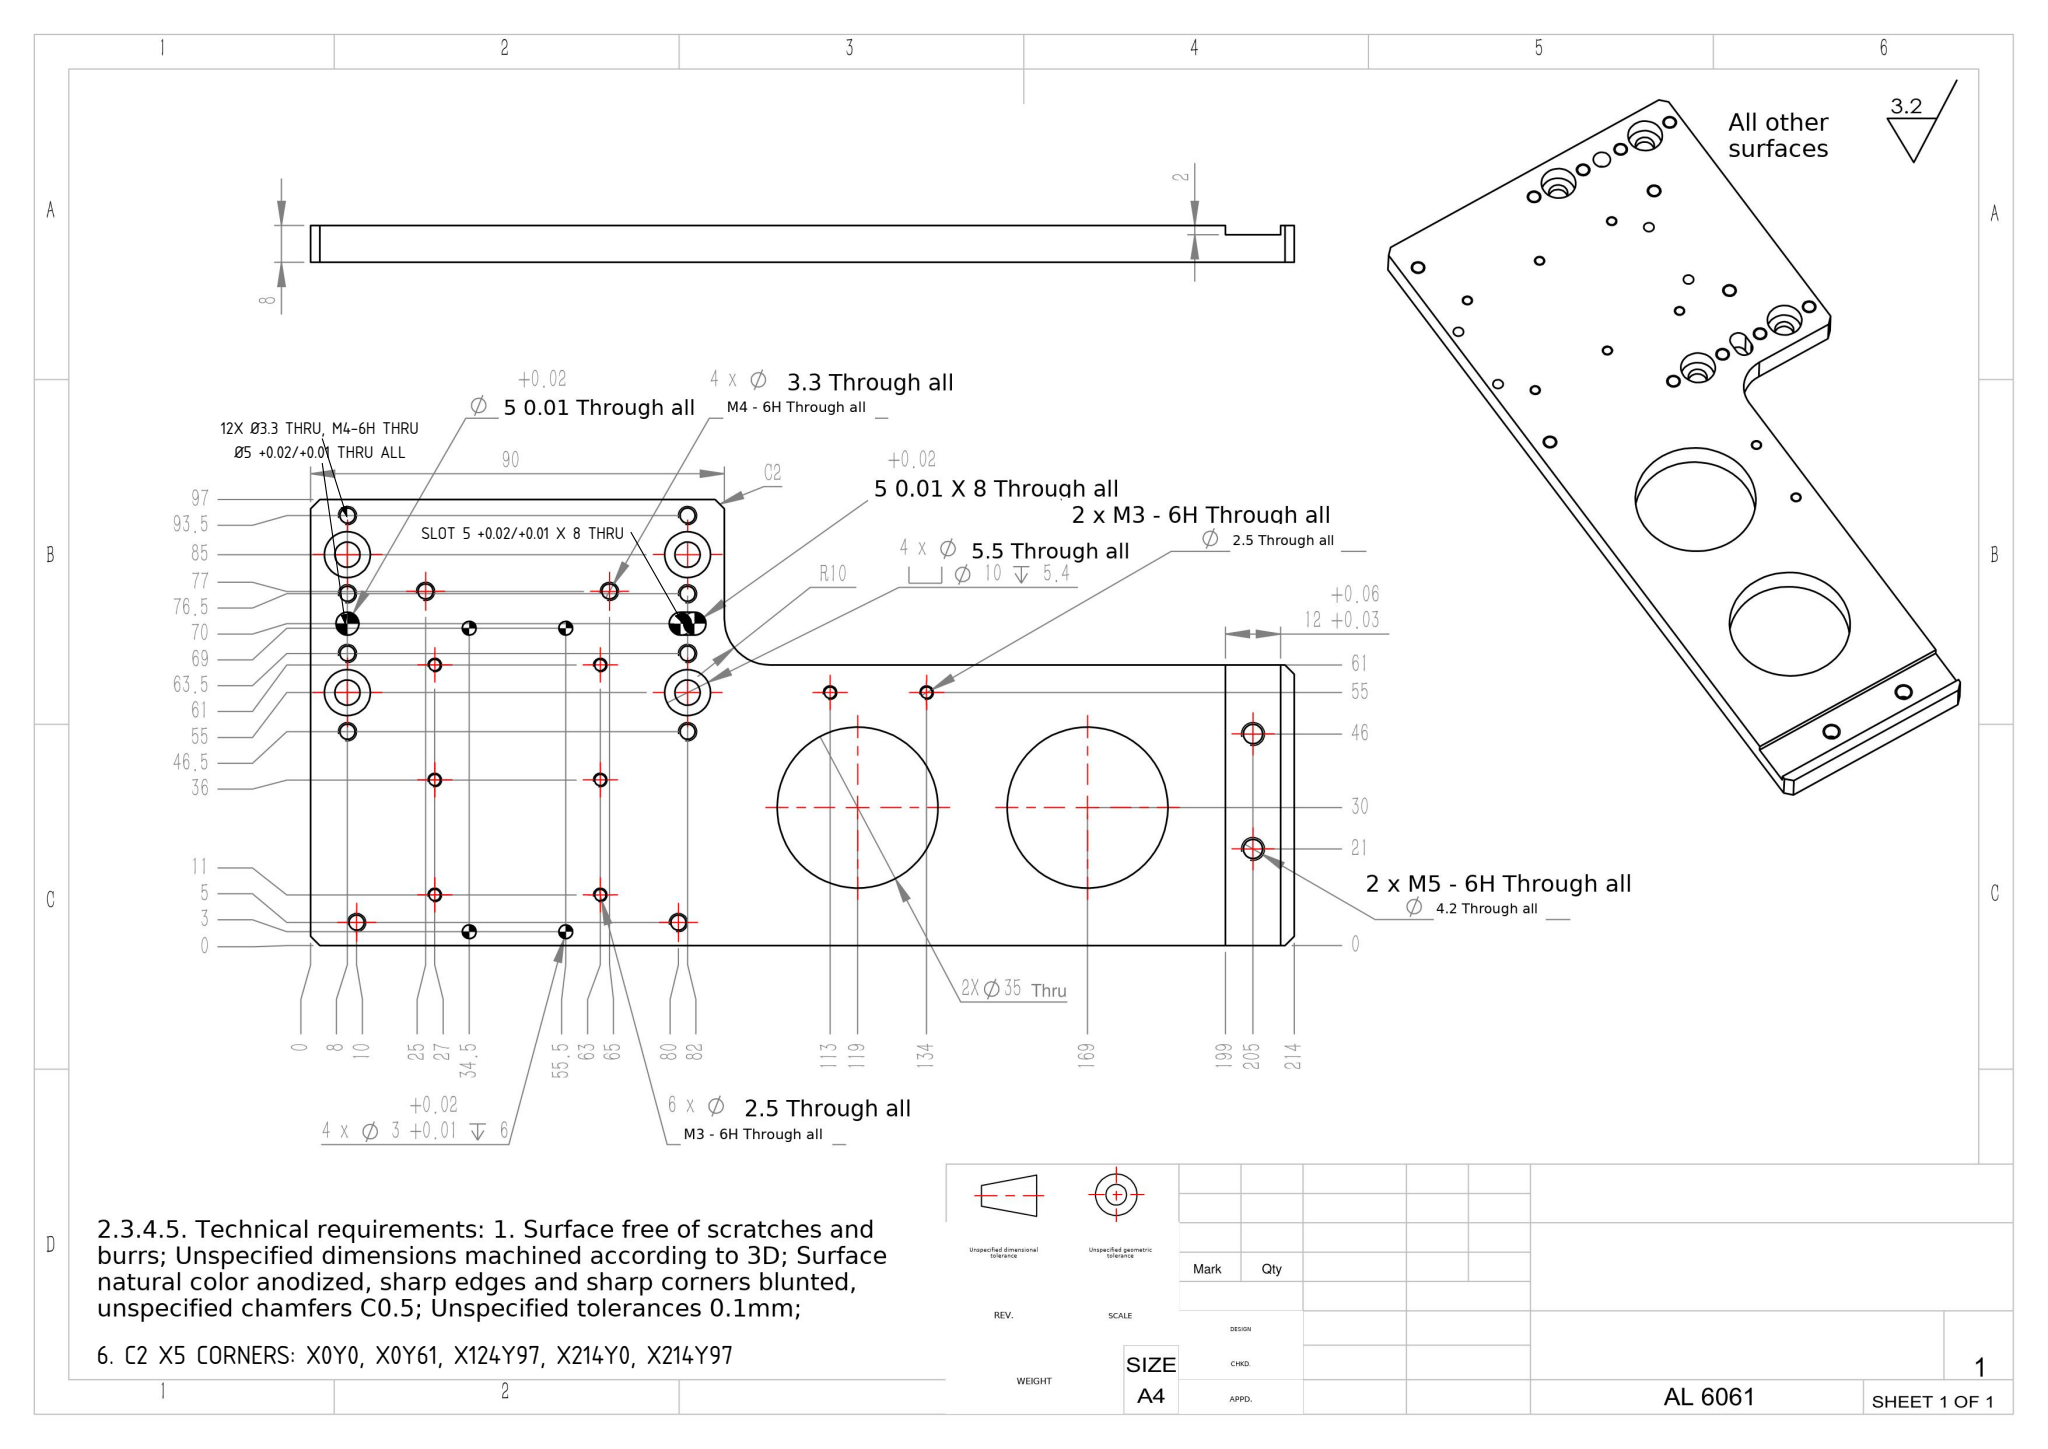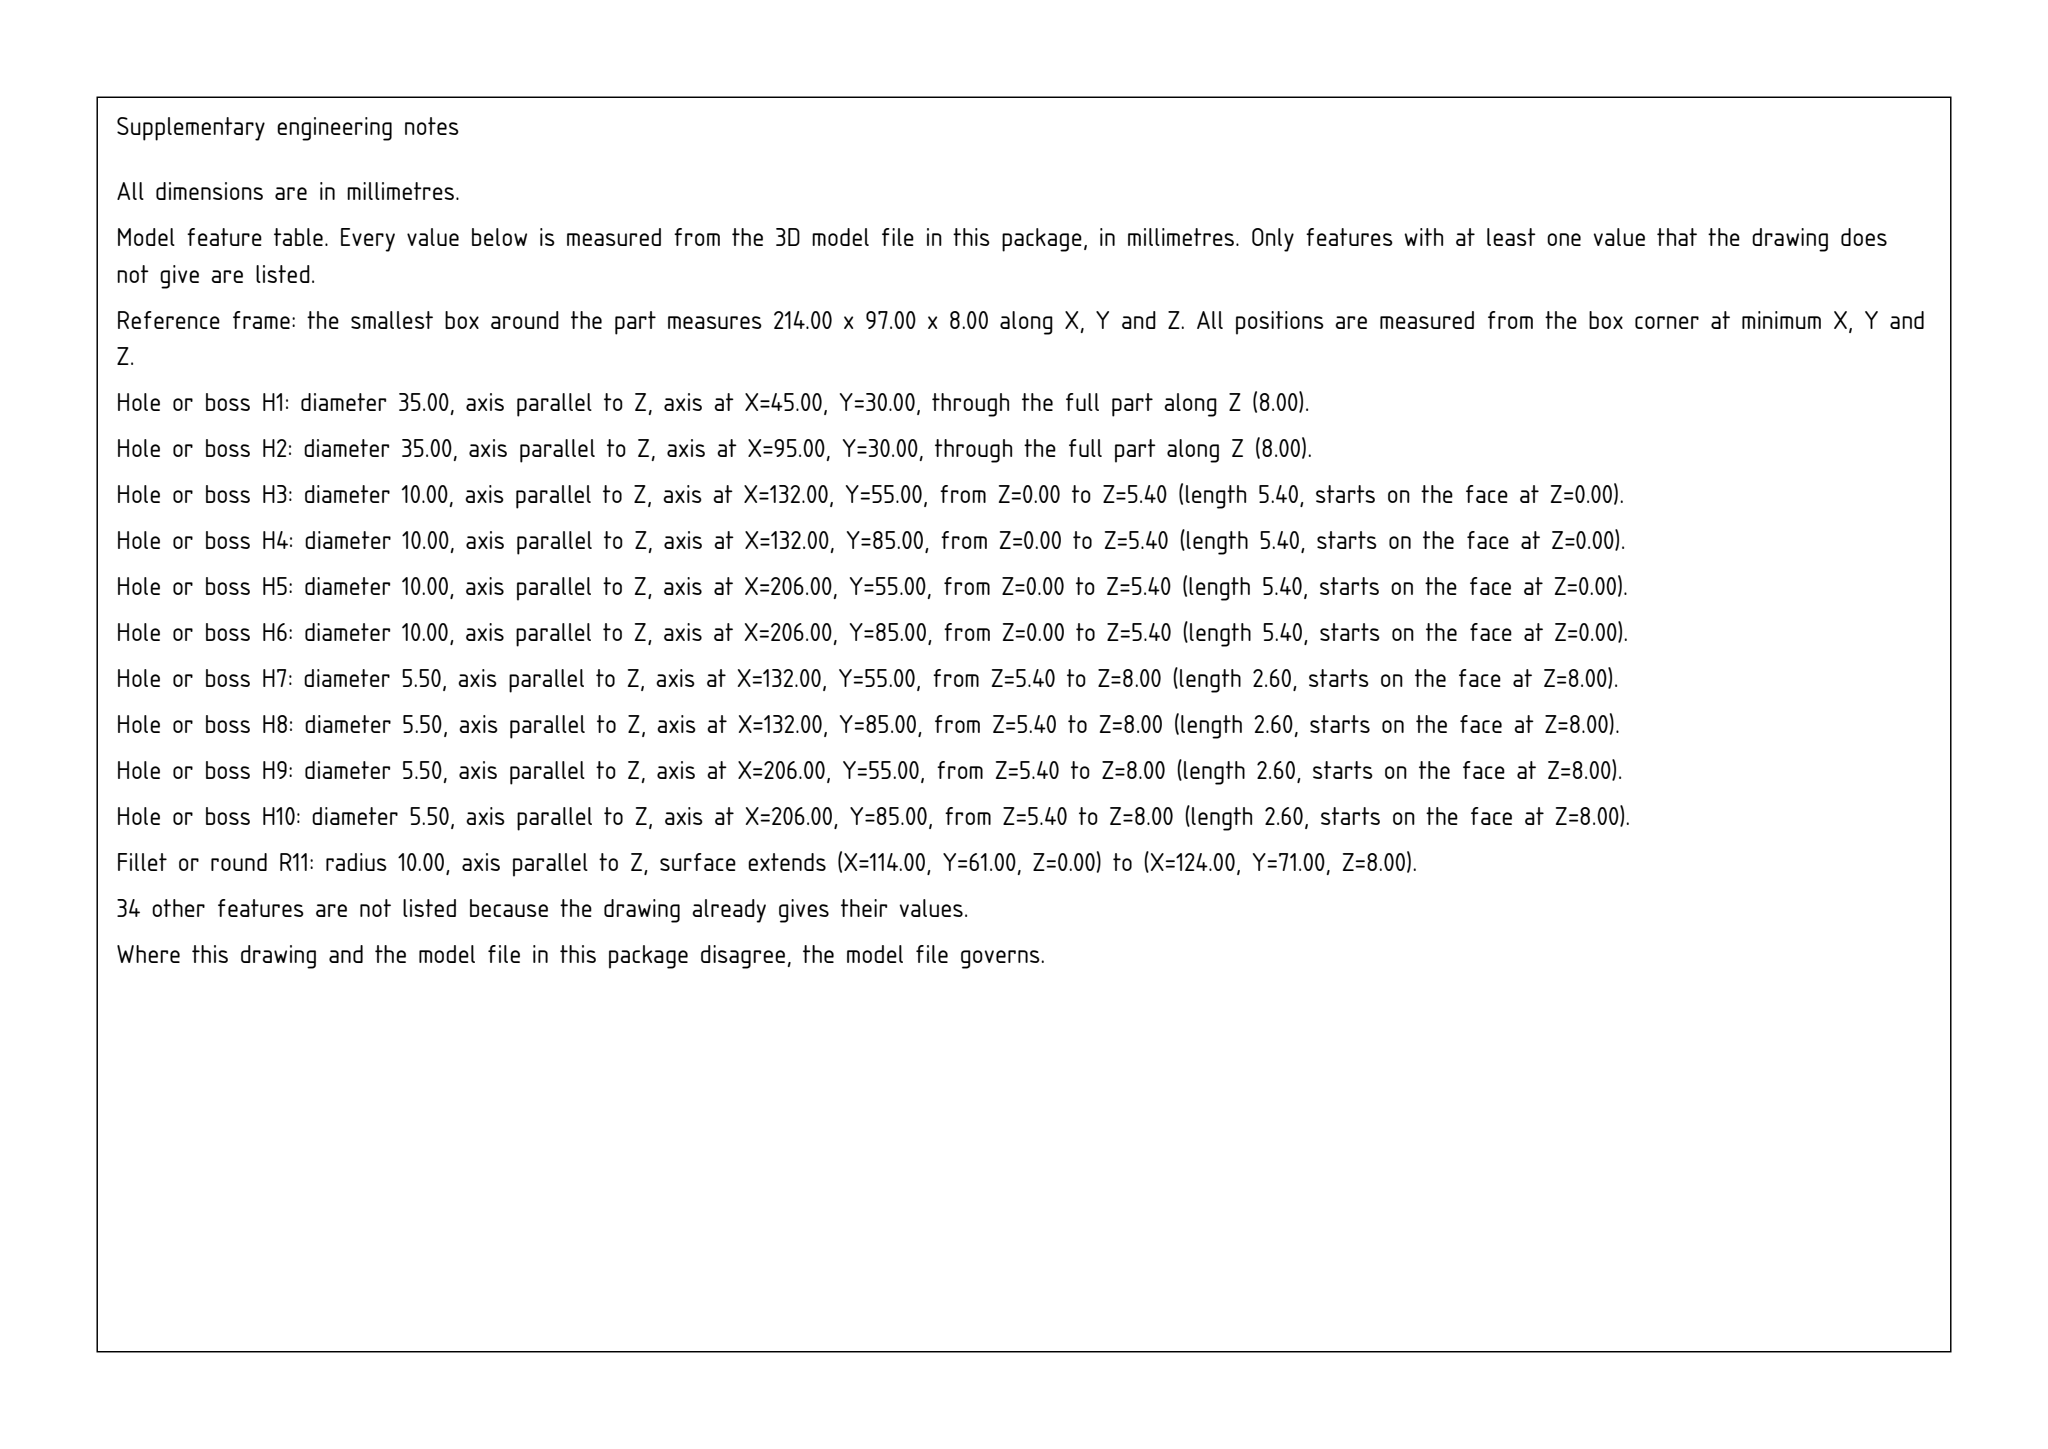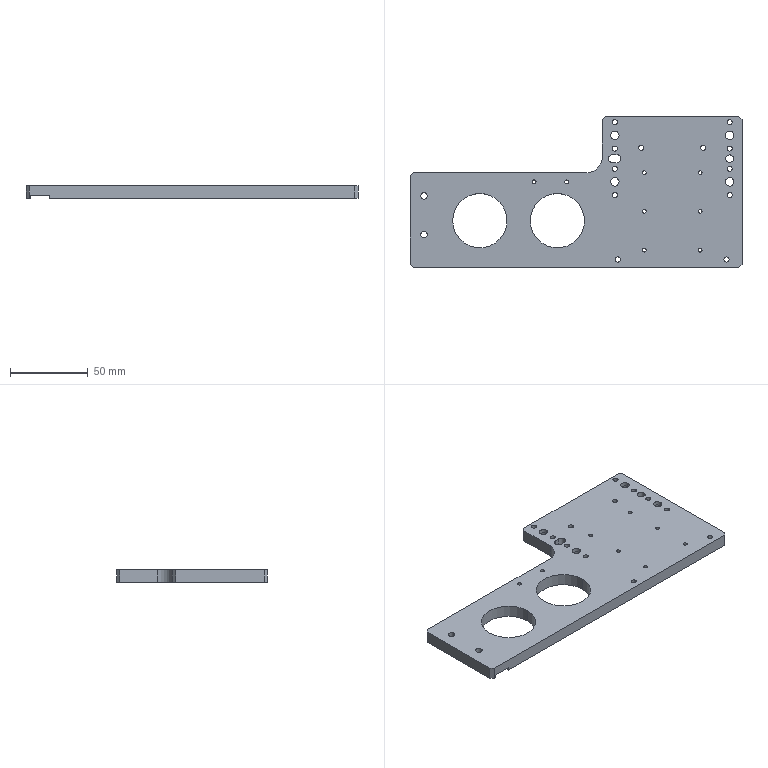Part | SolidWorks | mm | material AL 6061 | 1 solid | 109 faces | box 214 x 97 x 8 mm | volume 109729 mm3 | cylinder 78 | plane 23 | cone 8 | commonest cylinder face diameters 3.3 x24 2.5 x16 3 x8 10 x8 5.5 x8 5 x5 4.2 x4 35 x4
Drawing notes:
C2 X5 CORNERS: X0Y0, X0Y61, X124Y97, X214Y0, X214Y97 | from the solid: 5 inclined planes 45deg, size 2x2x8 at bbox_from [0,0,0], [0,59,0], [124,95,0], [212,0,0], [212,95,0]
1X Ø5 +0.02/+0.01 THRU ALL AT X206, Y70 | from the solid: hole/bore dia 5.0, axis z at [206.0, 70.0], from 0.0 to 8.0, 360 deg
SLOT 5 +0.02/+0.01 WIDE X 8 LG THRU ALL, CTR X132 Y70 | from the solid: two 180deg arcs dia 5 at [130.5,70] and [133.5,70] z0-8 + planes y=67.5 & y=72.5, x 130.5-133.5
12X Ø3.3 THRU ALL, M4-6H THRU ALL (NOT 4X) | from the solid: 12 holes dia 3.3 thru z0-8 at X132 Y46.5/63.5/76.5/93.5, X206 Y46.5/63.5/76.5/93.5, (134,5), (204,5), (149,77), (189,77)